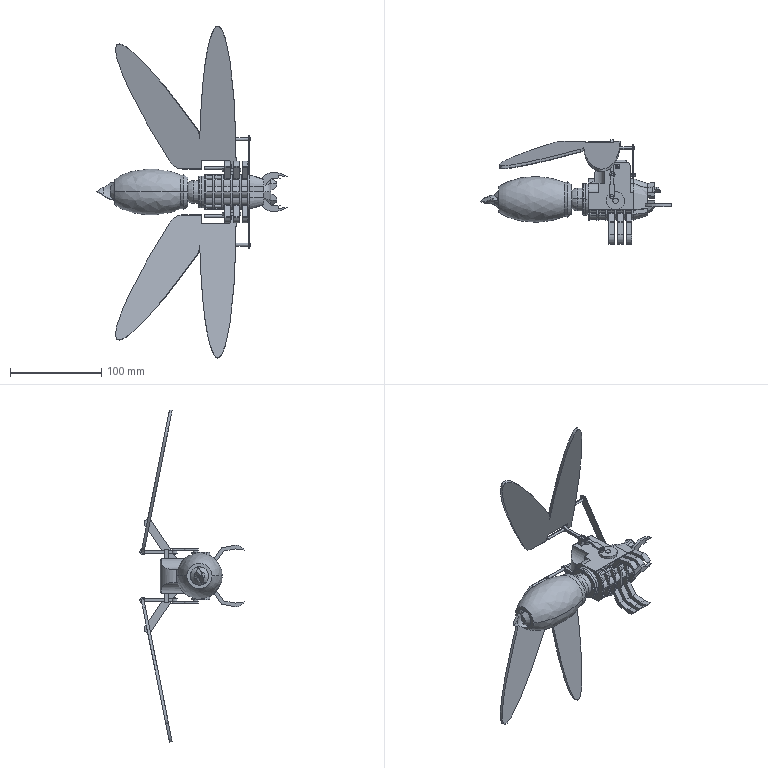Assembly | SolidWorks | mm | 29 component files | 29 solids | 825 faces | box 208.44 x 113.98 x 363.42 mm | volume 278620 mm3 | plane 355 | cylinder 285 | cone 155 | spline 18 | torus 8 | sphere 4 | commonest cylinder face diameters 3 x94 20 x42 6 x38 4 x24 2 x16 30 x14 40 x6 9 x6
Bill of materials:
10 | 1 |  | Thick circular disc with a through hole, a two-step cylindrical boss off-center on one face, and a larger cylindrical hub on the opposite face with a small radial cross hole.
1 | 1 |  | Hollow, barrel- or ellipsoid-shaped body with a through bore and a short cylindrical collar at one end.
11 | 2 |  | Thin flat plate outlined as two tapered, rounded lobes that meet at a common top edge, with a rectangular slot near that edge and a small thin pin sticking out from one side edge.
2 | 1 |  | Flanged tubular part: a circular flange with four bolt-pattern holes and a large central bore, a rounded bulged transition, and a smaller-diameter cylindrical tube section.
3 | 1 |  | Block-like body with a large cylindrical through bore and a rounded end. One side has five rib-like segments separated by slots, with small rods running along the length, and the top face has a small hole.
4 | 1 |  | Solid cylinder with a chamfered step down to a smaller section that continues into a curved, tapered, pointed tip with a hook-like profile.
5 | 1 | 45 | Pin-shaped part: a long slender cylindrical shaft on a thin circular flange, with a small two-step stub under the flange.
6 | 2 | 45 | Flat link plate of uniform thickness with a round hole at each end. One end has a wider rounded section, joined by a narrower neck to a ring-shaped eye at the other end.
7 | 2 |  | Slender straight bar with a ring eye at each end; the two eyes' hole axes appear to be about 90 degrees apart.
8 | 2 |  | Rectangular block with a stepped (L-shaped) profile. A rectangular slot under the taller portion forms two legs, and two round holes are on the top face.
9 | 1 |  | Plain cylindrical ring or sleeve with a concentric through bore and flat parallel end faces.
dj | 1 |  | Cylindrical body with a rounded edge at one end, from which a short boss and a smaller stepped shaft project. The shaft end appears to have a flat. Two small flat tabs with holes stick out from the opposite end.
Part12 | 2 | 45 | Thin flat elongated link/strap plate with fully rounded (semicircular) ends and one round through-hole near each end.
Part13 | 1 | 45 | Complex compact body: a tapered/flared housing section, a lobed end with two domed bumps, two curved C-shaped arms ending in barbed/notched tips, and a thin flat tab passing through the body.
Part14 | 6 | 45 | Bent flat bar of constant width and thickness with two bends. One end has an open circular hook (C-shaped slot); the other end is a curved, blade-like rounded end.
Part28 | 2 | 45 | Solid cylindrical pin with chamfered edges at both ends and flat end faces.
X2_5851659952369525_X0_b_X2_7120_X0 | 2 |  | Bevel-gear-like part: a conical toothed section with straight radial teeth on a cylindrical hub, and a central round through-bore.
Mates:
1. concentric | 1-1 face at (24.082, 8.534, 0) dir (-1, 0, 0) r 10 | 2-1 face at (21.329, 8.534, 0) dir (-1, 0, 0) r 10
2. coincident | 1-1 face at (21.329, 8.534, 0) dir (1, 0, 0) | 2-1 edge at (21.329, 8.534, 0) dir (1, 0, 0) r 10
3. concentric | 2-1 face at (21.329, 8.534, 0) dir (-1, 0, 0) r 8.5 | 3-1 face at (52.329, 8.534, 0) dir (1, 0, 0) r 15
4. coincident | 2-1 face at (36.329, 8.534, 0) dir (1, 0, 0) | 3-1 face at (36.329, 8.534, 0) dir (-1, 0, 0)
5. concentric | 1-1 face at (24.082, 8.534, 0) dir (-1, 0, 0) r 10 | 4-1 face at (-63.171, 8.534, 0) dir (1, 0, 0) r 10
6. coincident | 1-1 edge at (-58.671, 8.534, 0) dir (-1, 0, 0) r 10 | 4-1 edge at (-58.671, 8.534, 0) dir (1, 0, 0) r 10
7. concentric | 3-1 face at (69.329, 7.034, 72.062) dir (0, 0, -1) r 3 | 5-1 face at (69.329, 7.034, 27.062) dir (0, 0, -1) r 3
8. coincident | 3-1 plane at (36.329, 8.534, 0) dir (0, 0, -1) | assembly plane at (0, 0, 0) dir (0, 0, 1)
9. concentric | 5-1 face at (69.329, 7.034, 27.062) dir (0, 0, -1) r 3 | 9-1 face at (69.329, 7.034, -18.938) dir (0, 0, -1) r 3
10. coincident | 3-1 face at (19.479, 16.034, -18.938) dir (0, 0, -1) | 9-1 face at (69.329, 7.034, -18.938) dir (0, 0, 1)
11. coincident | 5-1 face at (69.329, 7.034, -22.938) dir (0, 0, 1) | 9-1 face at (69.329, 7.034, -22.938) dir (0, 0, -1)
12. concentric | 5-1 face at (65.208, 12.692, -29.938) dir (0, 0, 1) r 1.5 | 6-1 face at (65.208, 12.692, -29.938) dir (0, 0, 1) r 1.5
13. coincident | 5-1 face at (65.208, 12.692, -29.938) dir (0, 0, -1) | 6-1 face at (65.747, 35.686, -29.938) dir (0, 0, -1)
14. concentric | 6-1 face at (65.747, 35.686, -29.938) dir (0, 0, 1) r 1.5 | 7-1 face at (65.747, 35.686, -34.938) dir (0, 0, 1) r 1.5
15. coincident | 6-1 face at (65.747, 35.686, -27.938) dir (0, 0, 1) | 7-1 face at (65.747, 70.686, -27.938) dir (0, 0, -1)
16. coincident | 3-1 face at (19.479, 16.034, -18.938) dir (0, 0, -1) | 8-1 face at (68.747, 46.914, -18.938) dir (0, 0, 1)
17. parallel | 3-1 face at (46.144, 56.558, 75.323) dir (-1, 0, 0) | 8-1 face at (62.747, 46.914, -18.938) dir (-1, 0, 0)
18. width | 8-1 face at (68.747, 46.914, -18.938) dir (1, 0, 0) | 8-1 face at (62.747, 46.914, -18.938) dir (-1, 0, 0) | 3-1 face at (46.144, 56.558, 75.323) dir (-1, 0, 0) | 3-1 face at (85.35, 56.558, 75.323) dir (1, 0, 0)
19. concentric | 5-1 face at (69.329, 7.034, 27.062) dir (0, 0, -1) r 3 | 10-1 face at (69.329, 7.034, 46.938) dir (0, 0, -1) r 3
20. coincident | 3-1 face at (19.479, 16.034, 18.938) dir (0, 0, 1) | 10-1 face at (69.329, 7.034, 18.938) dir (0, 0, -1)
21. coincident | 7-1 face at (67.247, 70.686, -24.938) dir (1, 0, 0) | 8-1 face at (67.247, 46.914, -28.938) dir (-1, 0, 0)
22. concentric | 3-1 face at (71.247, 44.414, -13.938) dir (0, 0, -1) r 1 | 8-1 face at (71.247, 44.414, -16.938) dir (0, 0, -1) r 1
23. concentric | 7-1 face at (67.247, 70.686, -26.438) dir (-1, 0, 0) r 1.5 | 11-1 face at (74.247, 70.686, -26.438) dir (-1, 0, 0) r 1.5
24. concentric | 11-1 face at (90.247, 64.493, -57.666) dir (-1, 0, 0) r 1.5 | Part12-1 face at (89.229, 64.493, -57.666) dir (-1, 0, 0) r 1.5
25. concentric | 3-1 face at (91.35, 35.432, -14.497) dir (-1, 0, 0) r 1.5 | Part12-1 face at (89.229, 35.432, -14.497) dir (-1, 0, 0) r 1.5
26. concentric | 10-1 face at (65.208, 12.692, 29.938) dir (0, 0, -1) r 1.5 | 6-3 face at (65.208, 12.692, 27.938) dir (0, 0, 1) r 1.5
27. coincident | 7-1 face at (67.247, 70.686, -24.938) dir (1, 0, 0) | 11-1 face at (67.247, 70.686, -26.438) dir (-1, 0, 0)
28. concentric | 3-1 face at (37.087, -7.312, -15.655) dir (1, 0, 0) r 1.5 | Part14-1 face at (87.329, -7.312, -15.655) dir (-1, 0, 0) r 1.5
29. coincident | 3-1 face at (87.329, -3.966, 2.367) dir (-1, 0, 0) | Part14-1 face at (87.329, -2.38, 5.911) dir (1, 0, 0)
30. concentric | 2-1 face at (21.329, 8.534, 0) dir (-1, 0, 0) r 8.5 | dj-1 face at (49.669, 8.534, 0) dir (-1, 0, 0) r 8.5
31. concentric | dj-1 face at (63.669, 8.534, 0) dir (-1, 0, 0) r 3 | X2_5851659952369525_X0_b_X2_7120_X0-3 face at (68.469, 8.534, 0) dir (1, 0, 0) r 3
32. coincident | dj-1 face at (63.669, 8.534, 0) dir (1, 0, 0) | X2_5851659952369525_X0_b_X2_7120_X0-3 face at (63.669, 11.025, -0.2111) dir (1, 0, 0)
33. concentric | 5-1 face at (69.329, 7.034, 27.062) dir (0, 0, -1) r 3 | X2_5851659952369525_X0_b_X2_7120_X0-4 face at (69.329, 7.034, 0.5018) dir (0, 0, 1) r 3
34. gear | X2_5851659952369525_X0_b_X2_7120_X0-4 face at (69.329, 7.034, 0.5018) dir (0, 0, 1) r 6 | X2_5851659952369525_X0_b_X2_7120_X0-3 face at (68.469, 8.534, 0) dir (1, 0, 0) r 6
35. distance | 9-1 face at (69.329, 7.034, -18.938) dir (0, 0, 1) | X2_5851659952369525_X0_b_X2_7120_X0-4 face at (69.329, 7.034, -12.898) dir (0, 0, -1)
36. distance | dj-1 face at (49.669, 8.534, 0) dir (1, 0, 0) | 2-1 face at (36.329, 8.534, 0) dir (1, 0, 0)
37. coincident | 10-1 plane at (69.329, 7.034, 22.938) dir (0.8083, 0.5888, 0) | X2_5851659952369525_X0_b_X2_7120_X0-4 plane at (69.329, 7.034, 0.5018) dir (0.8083, 0.5888, 0)
38. concentric | 6-3 face at (65.747, 35.686, 27.938) dir (0, 0, 1) r 1.5 | Part28-1 face at (65.747, 35.686, 29.938) dir (0, 0, -1) r 1.5
39. coincident | 6-3 face at (65.747, 35.686, 29.938) dir (0, 0, 1) | Part28-1 face at (65.747, 35.686, 29.938) dir (0, 0, 1)
40. concentric | 7-1 face at (65.747, 35.686, -34.938) dir (0, 0, 1) r 1.5 | Part28-2 face at (65.747, 35.686, -23.938) dir (0, 0, -1) r 1.5
41. coincident | 6-1 face at (65.747, 35.686, -29.938) dir (0, 0, -1) | Part28-2 face at (65.747, 35.686, -29.938) dir (0, 0, -1)